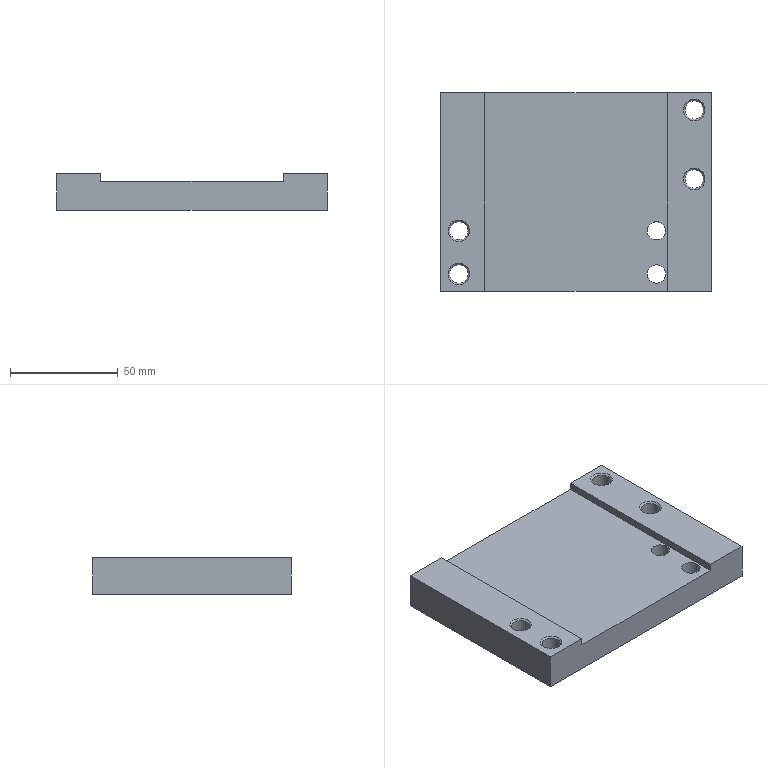Component | NX | CLHKJG_01_BASE | 1 solid | 26 faces | volume 163603 mm3 | plane 10 | cone 10 | cylinder 6 | commonest cylinder face diameters 8.5 x6